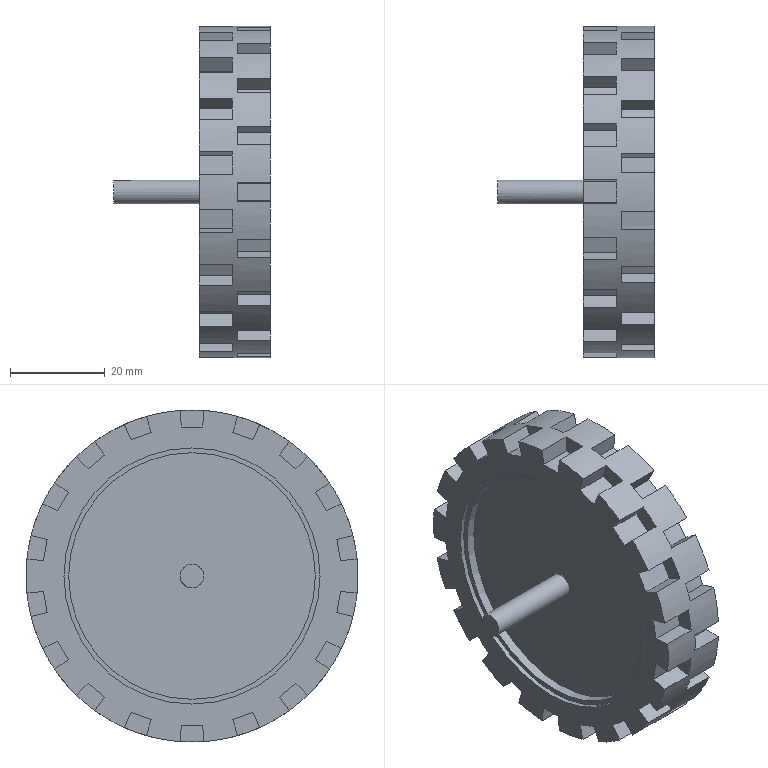Component | NX | MIRRORED_WHEEL | 1 solid | 153 faces | volume 47782 mm3 | plane 149 | cylinder 4 | commonest cylinder face diameters 70 x1 54 x1 52 x1 5 x1